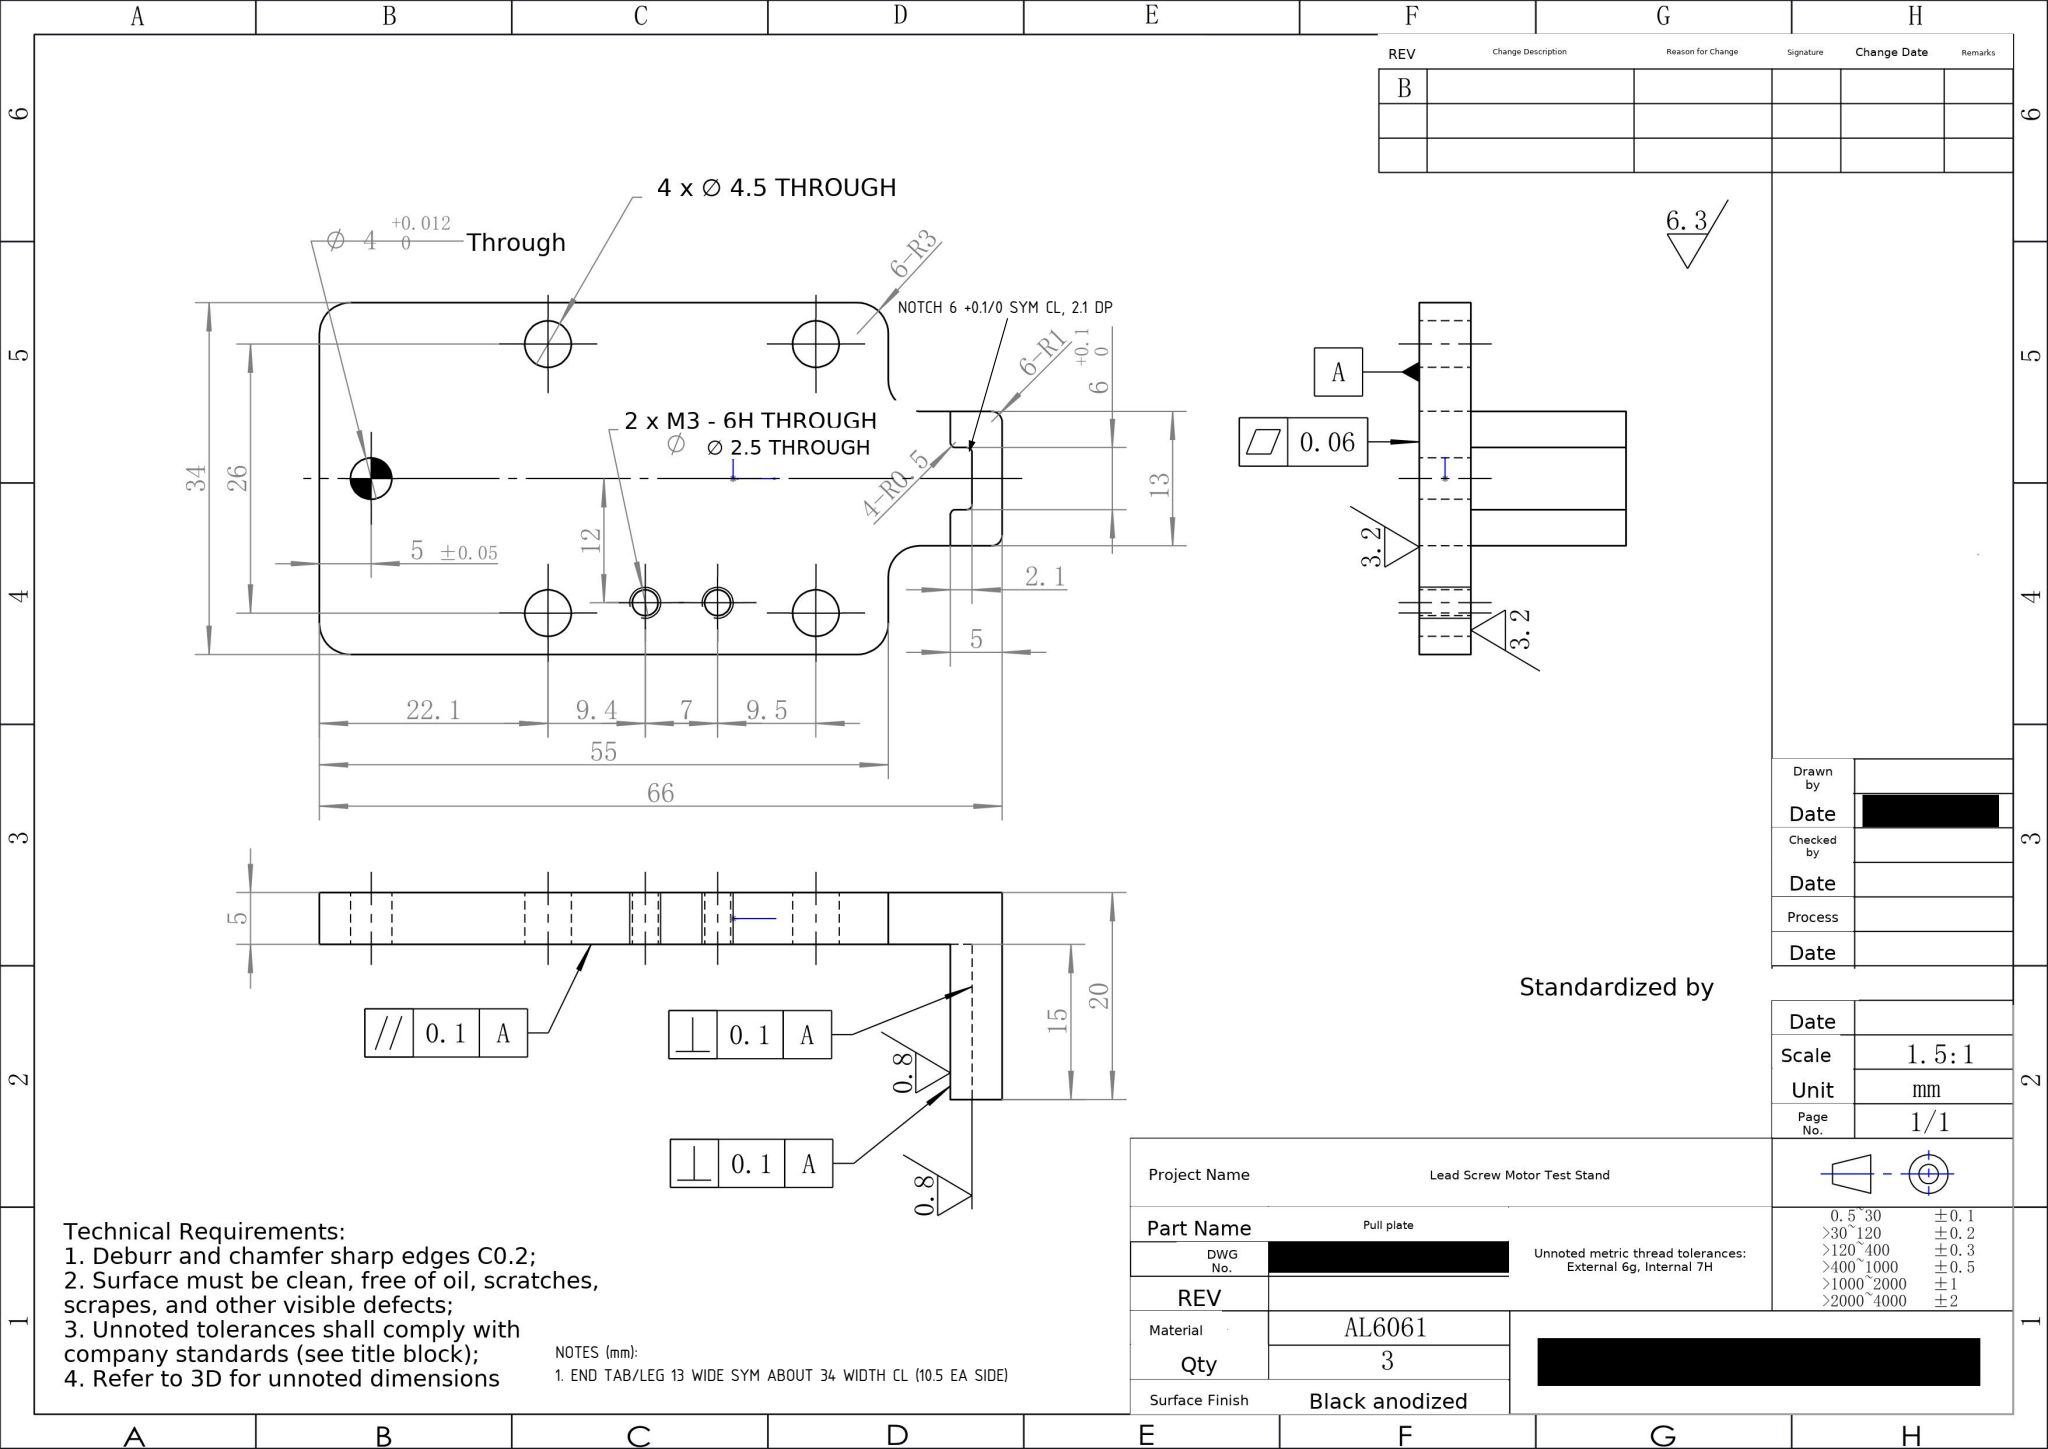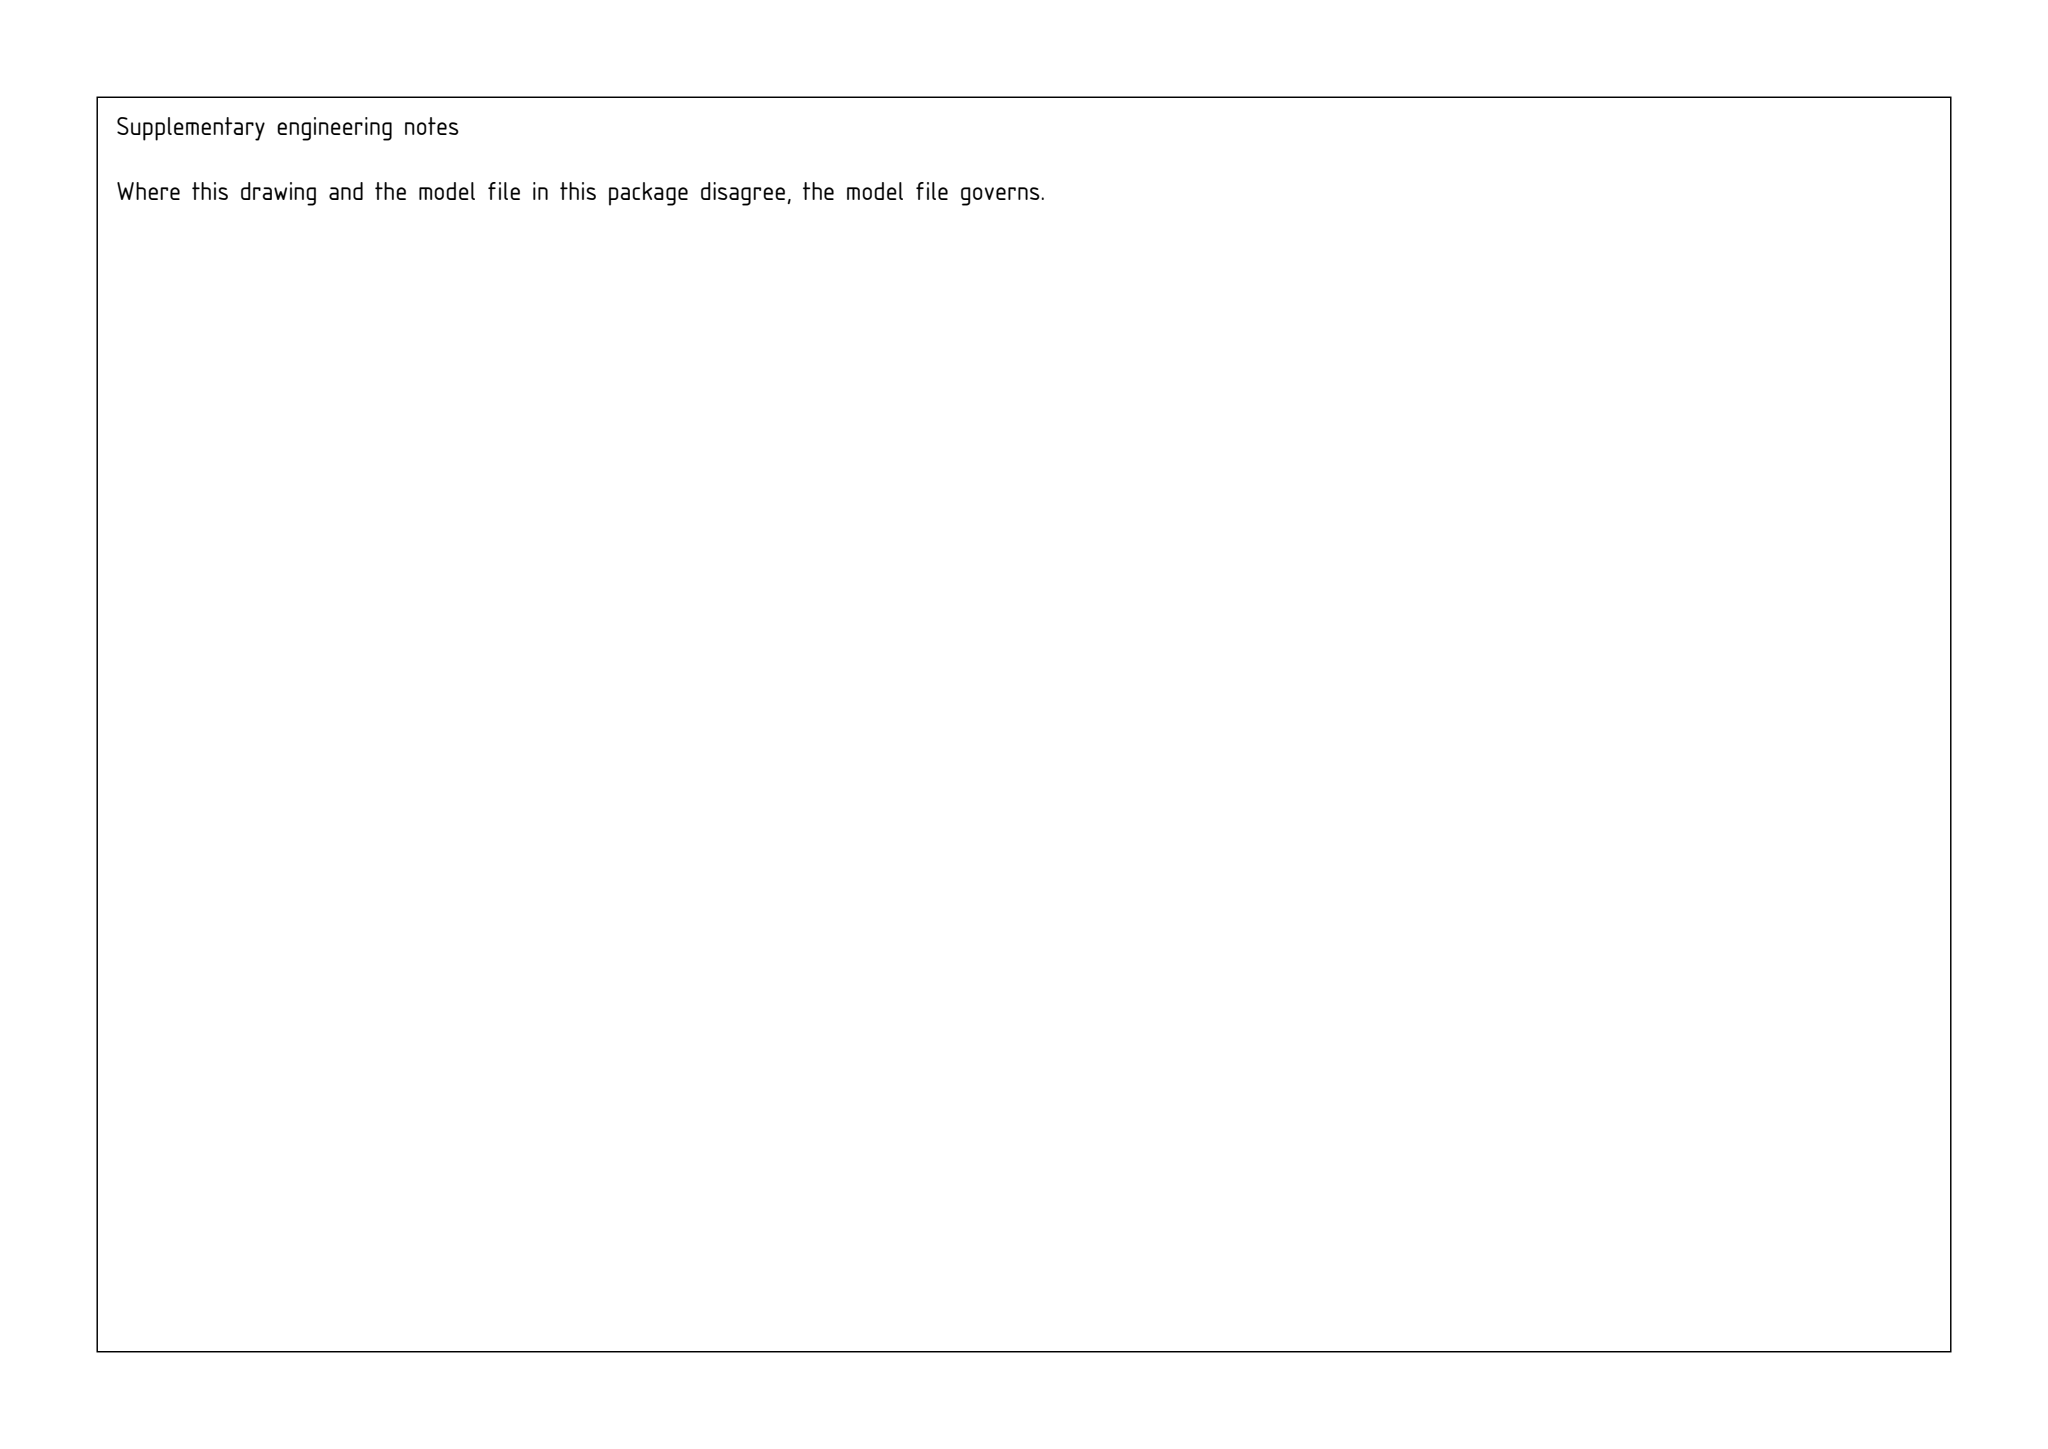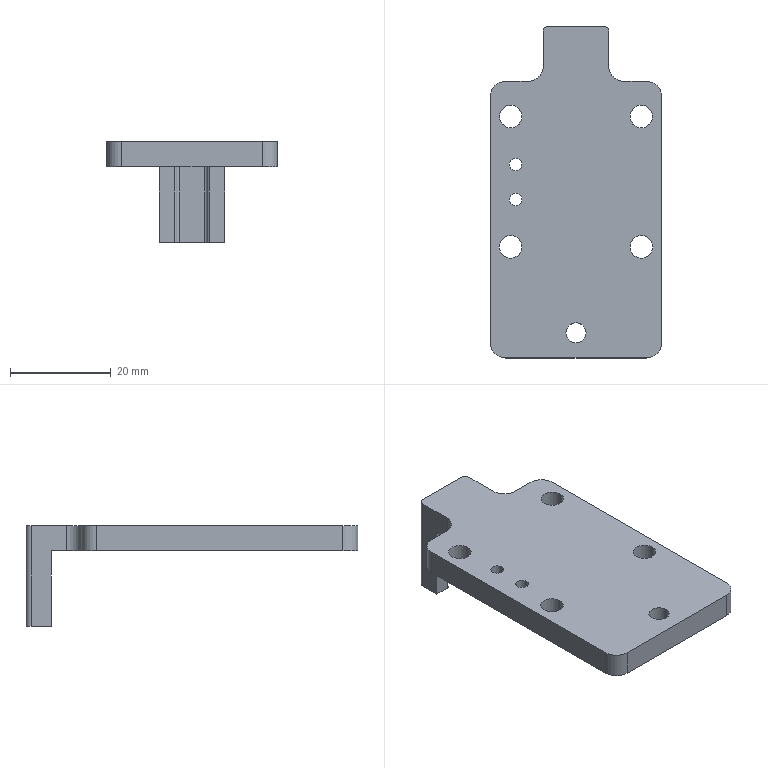Part | SolidWorks | mm | material AL6061 | 1 solid | 42 faces | box 34 x 66 x 20 mm | volume 10393 mm3 | cylinder 26 | plane 16 | commonest cylinder face diameters 4.5 x8 6 x6 2.5 x4 1 x4 4 x2 2 x2
Drawing notes:
END TAB/LEG 13 WIDE SYM ABOUT 34 WIDTH CL (10.5 EA SIDE) | from the solid: Tab faces x=10.5 & x=23.5 (13 wide) in bbox x=34, centered on CL x=17
NOTCH 6 +0.1/0 SYM ABOUT CL, 2.1 DP, THRU FULL 15 LEG, INNER FACE 5 FROM END FACE | from the solid: Notch walls x=14 & x=20 (CL 17); y=61 to 63.1 = 2.1 DP; 4-R0.5 corners 15 long; leg y=61 to 66 = 5 thk
build123d program:
from build123d import *

# Parameters (mm, degrees)
SKETCH1_W                = 34
SKETCH1_H                = 50
BOSS_EXTRUDE1_DEPTH      = 2.5
SKETCH2_W                = 10.5
SKETCH2_H                = 10
CUT_EXTRUDE1_DEPTH       = 31.643
SKETCH3_W                = 13
SKETCH3_H                = 4
BOSS_EXTRUDE2_DEPTH      = 15
SKETCH4_R                = 2.05
CUT_EXTRUDE2_DEPTH       = 12
FILLET1_R                = 1
M4_CLEARANCE_HOLE1_D     = 4.5
M3_TAPPED_HOLE1_D        = 2.5
SKETCH11_W               = 34
SKETCH11_H               = 15
BOSS_EXTRUDE3_DEPTH      = 5
F_4_0_4_DIAMETER_HOLE1_D = 4
FILLET3_R                = 3
SKETCH14_W               = 13
SKETCH14_H               = 20
BOSS_EXTRUDE4_DEPTH      = 1
SKETCH15_W               = 6
SKETCH15_H               = 4.2
CUT_EXTRUDE3_DEPTH       = 15
FILLET4_R                = 0.5
FILLET5_R                = 1


with BuildPart() as part:
    # Sketch1 → Boss-Extrude1 (new, symmetric)
    with BuildSketch(Plane.XY):
        Rectangle(SKETCH1_W, SKETCH1_H)
    extrude(amount=BOSS_EXTRUDE1_DEPTH, both=True)

    # Sketch2 → Cut-Extrude1 (cut, through all)
    with BuildSketch(Plane.XY.offset(2.5)):
        with Locations((-11.75, 20)):
            Rectangle(SKETCH2_W, SKETCH2_H)
        with Locations((11.75, 20)):
            Rectangle(SKETCH2_W, SKETCH2_H)
    extrude(amount=-CUT_EXTRUDE1_DEPTH, mode=Mode.SUBTRACT)

    # Sketch3 → Boss-Extrude2 (add)
    with BuildSketch(Plane(origin=(0, 0, -2.5), x_dir=(-1, 0, 0), z_dir=(0, 0, -1))):
        with Locations((0, 23)):
            Rectangle(SKETCH3_W, SKETCH3_H)
    extrude(amount=BOSS_EXTRUDE2_DEPTH)

    # Sketch4 → Cut-Extrude2 (cut)
    with BuildSketch(Plane(origin=(0, 0, -17.5), x_dir=(-1, 0, 0), z_dir=(0, 0, -1))):
        with Locations((0, 21)):
            Circle(SKETCH4_R)
    extrude(amount=-CUT_EXTRUDE2_DEPTH, mode=Mode.SUBTRACT)

    # Fillet1
    fillet1_edges = [part.edges().sort_by_distance(p)[0] for p in [
        (2.05, 21, -11.5),
        (-2.05, 21, -11.5),
    ]]
    fillet(fillet1_edges, radius=FILLET1_R)

    # M4 Clearance Hole1 (through all)
    with Locations(Plane(origin=(0, 0, -2.5), x_dir=(-1, 0, 0), z_dir=(0, 0, -1))):
        with Locations((-13, -17.9), (13, -17.9), (13, 8), (-13, 8)):
            Hole(M4_CLEARANCE_HOLE1_D / 2)

    # M3 Tapped Hole1 (through all)
    with Locations(Plane(origin=(0, 0, -2.5), x_dir=(-1, 0, 0), z_dir=(0, 0, -1))):
        with Locations((12, -8.5), (12, -1.5)):
            Hole(M3_TAPPED_HOLE1_D / 2)

    # Sketch11 → Boss-Extrude3 (add, through all)
    with BuildSketch(Plane(origin=(0, 0, -2.5), x_dir=(-1, 0, 0), z_dir=(0, 0, -1))):
        with Locations((0, -32.5)):
            Rectangle(SKETCH11_W, SKETCH11_H)
    extrude(amount=-BOSS_EXTRUDE3_DEPTH)

    # 4.0 _4_ Diameter Hole1 (through all)
    with Locations(Plane(origin=(0, 0, -2.5), x_dir=(-1, 0, 0), z_dir=(0, 0, -1))):
        with Locations((0, -35)):
            Hole(F_4_0_4_DIAMETER_HOLE1_D / 2)

    # Fillet3
    fillet3_edges = [part.edges().sort_by_distance(p)[0] for p in [
        (17, -40, 0),
        (-17, -40, 0),
        (-17, 15, 0),
        (-6.5, 15, 0),
        (17, 15, 0),
        (6.5, 15, 0),
    ]]
    fillet(fillet3_edges, radius=FILLET3_R)

    # Sketch14 → Boss-Extrude4 (add)
    with BuildSketch(Plane(origin=(0, 25, 0), x_dir=(1, 0, 0), z_dir=(0, 1, 0))):
        with Locations((0, 7.5)):
            Rectangle(SKETCH14_W, SKETCH14_H)
    extrude(amount=BOSS_EXTRUDE4_DEPTH)

    # Sketch15 → Cut-Extrude3 (cut)
    with BuildSketch(Plane(origin=(0, 0, -17.5), x_dir=(-1, 0, 0), z_dir=(0, 0, -1))):
        with Locations((0, 21)):
            Rectangle(SKETCH15_W, SKETCH15_H)
    extrude(amount=-CUT_EXTRUDE3_DEPTH, mode=Mode.SUBTRACT)

    # Fillet4
    fillet4_edges = [part.edges().sort_by_distance(p)[0] for p in [
        (3, 21, -10),
        (-3, 21, -10),
        (-3, 23.1, -10),
        (3, 23.1, -10),
    ]]
    fillet(fillet4_edges, radius=FILLET4_R)

    # Fillet5
    fillet5_edges = [part.edges().sort_by_distance(p)[0] for p in [
        (6.5, 26, -7.5),
        (-6.5, 26, -7.5),
    ]]
    fillet(fillet5_edges, radius=FILLET5_R)


solid = part.part